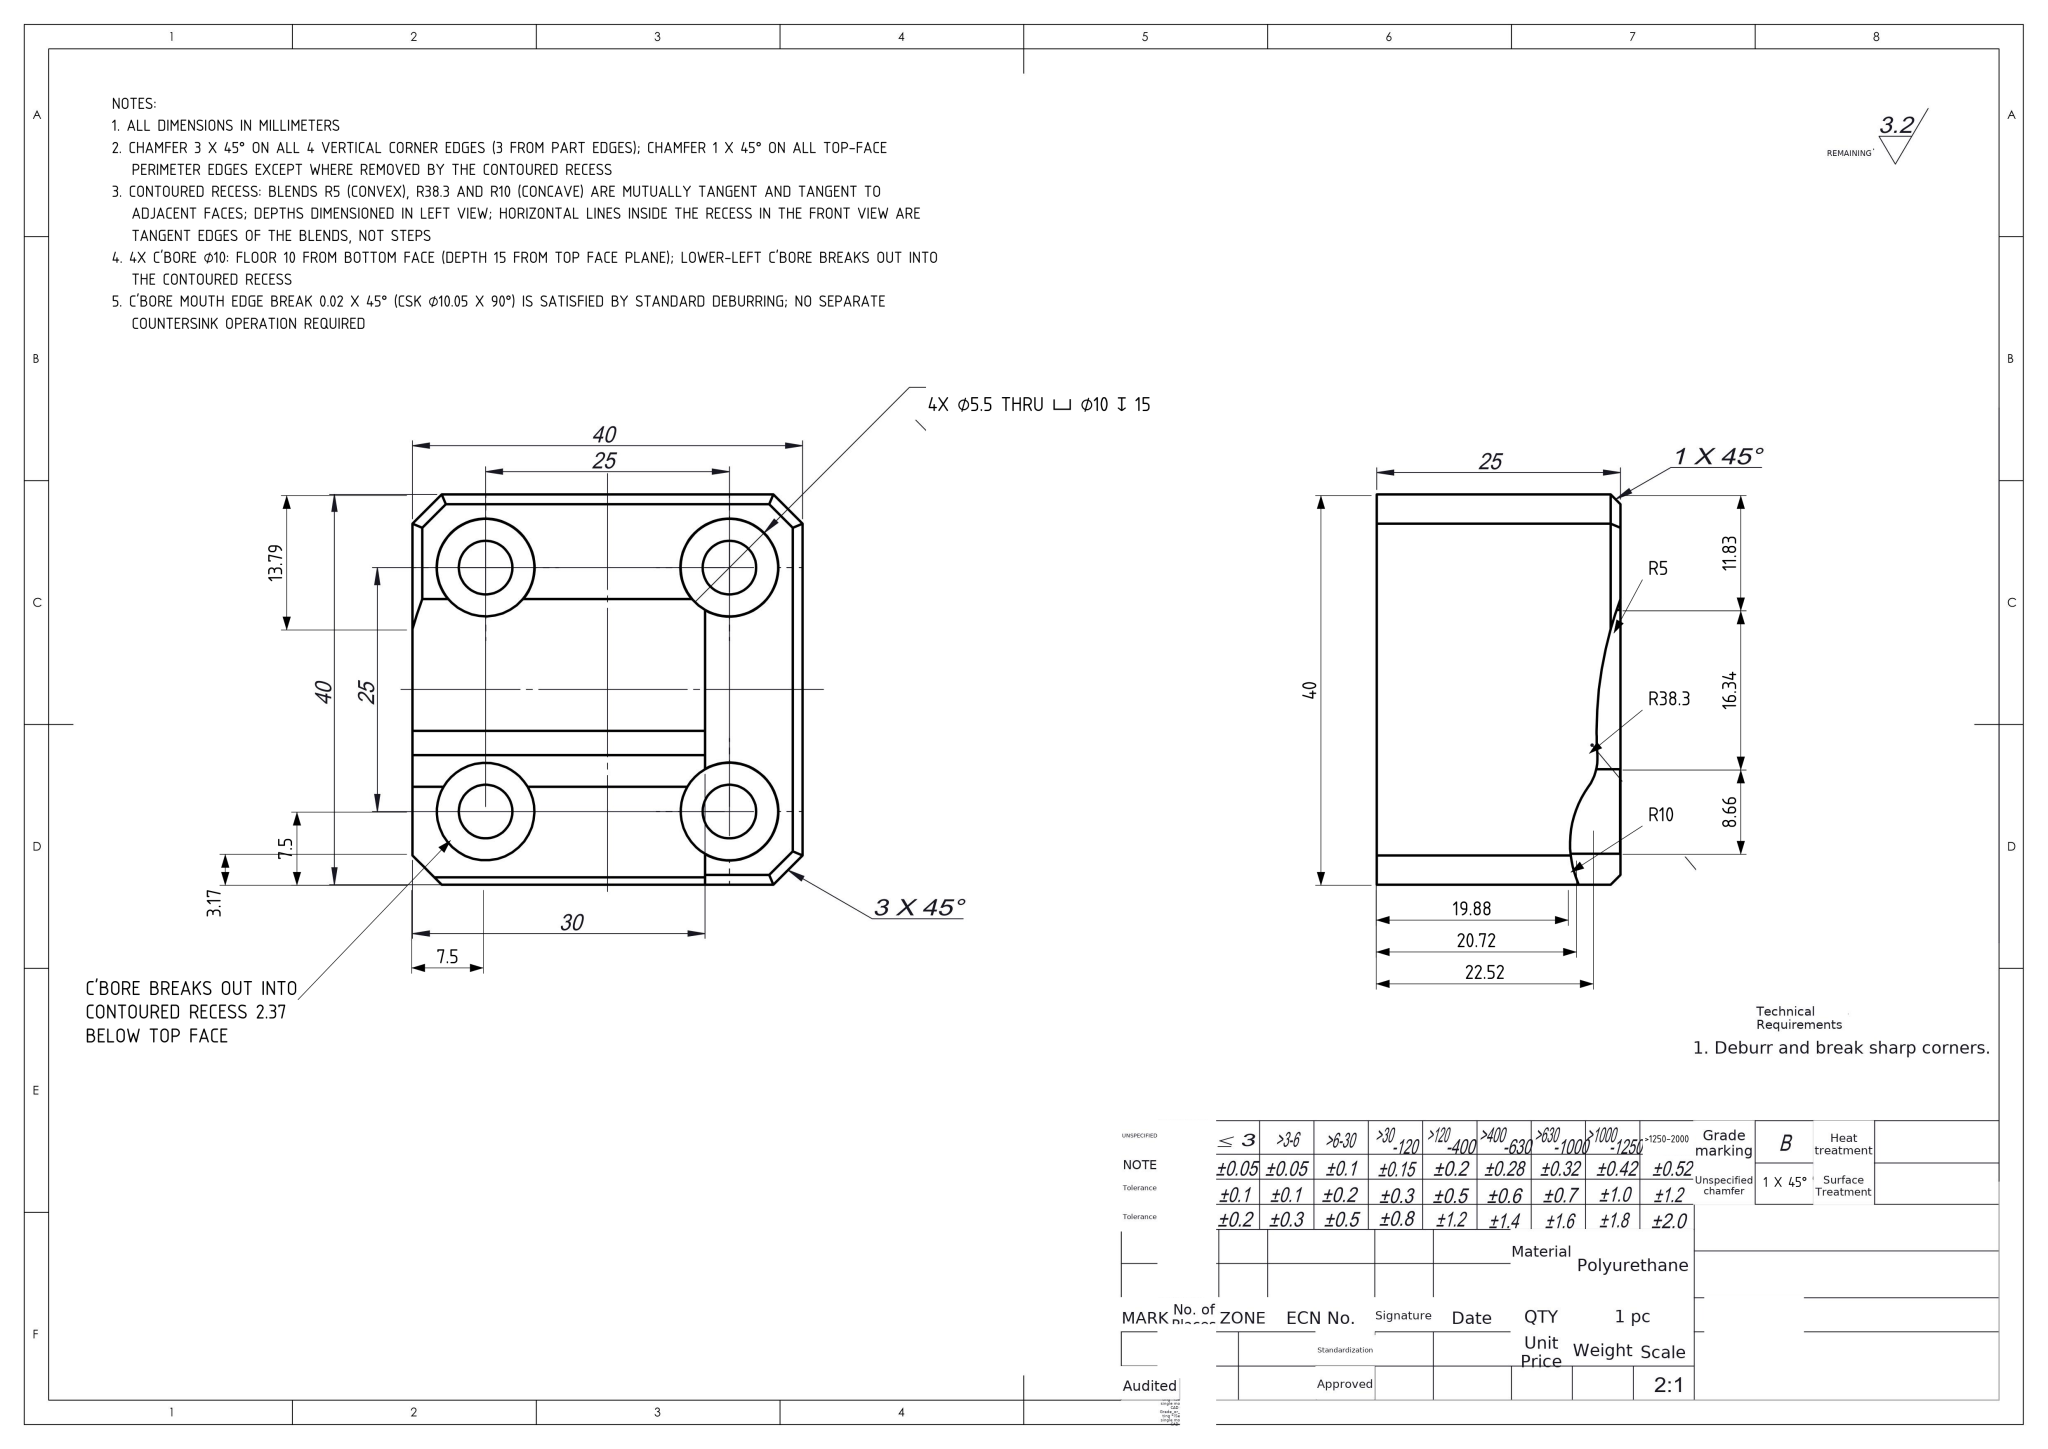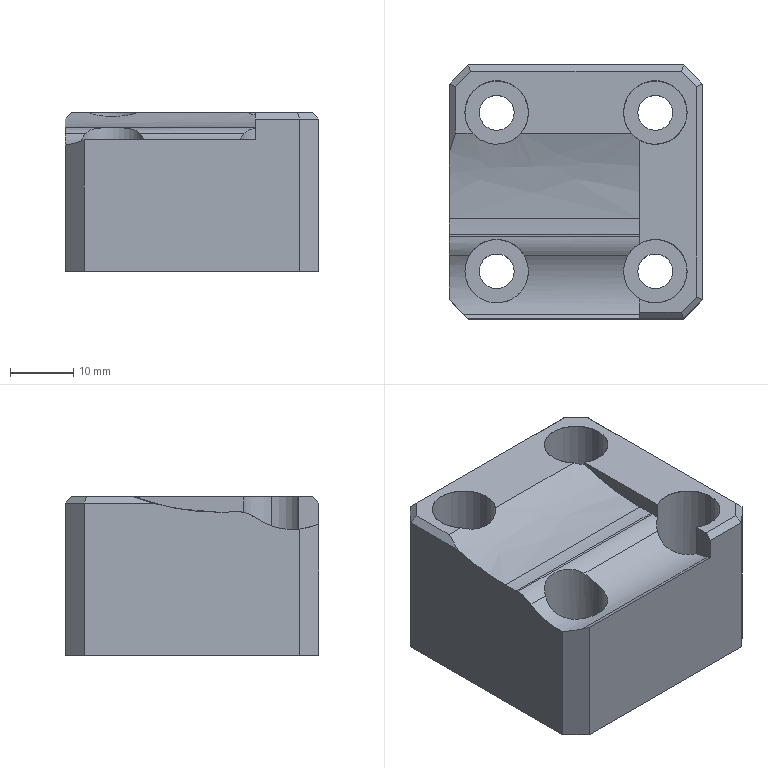Part | NX | mm | 1 solid | 53 faces | box 40 x 40 x 25 mm | volume 31753 mm3 | plane 23 | cylinder 20 | cone 8 | spline 2 | commonest cylinder face diameters 10 x10 5.5 x8 20 x1 76.607 x1